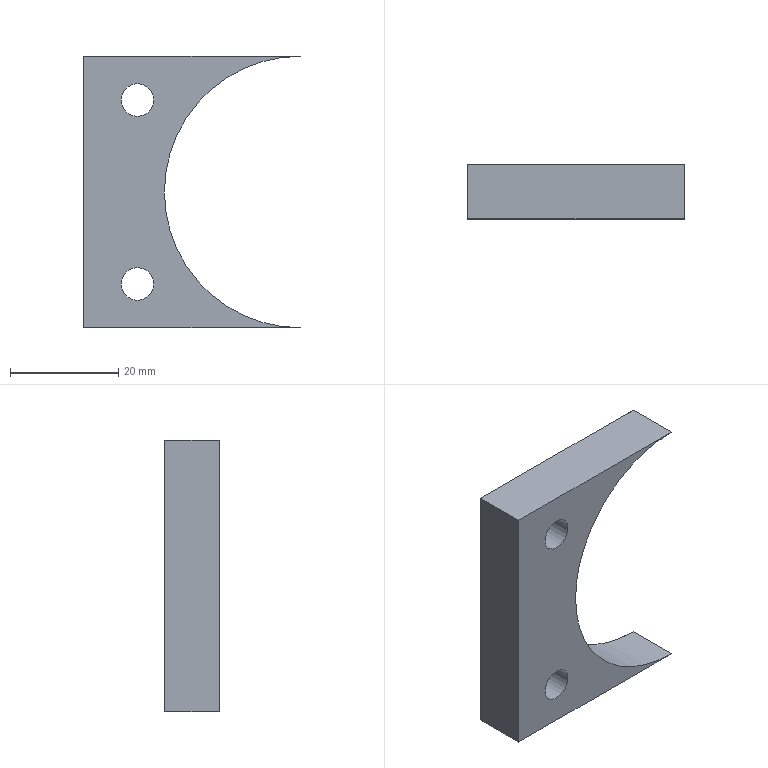Component | NX | GUIDEING_PLATE_2 | 1 solid | 10 faces | box 40 x 10 x 50.2 mm | volume 9461 mm3 | plane 5 | cylinder 3 | cone 2 | commonest cylinder face diameters 6 x2 50.2 x1
STEP:
#1=CARTESIAN_POINT('',(0.,0.,0.));
#2=DIRECTION('',(0.,0.,1.));
#3=DIRECTION('',(1.,0.,0.));
#4=AXIS2_PLACEMENT_3D('',#1,#2,#3);
#5=CARTESIAN_POINT('',(-114.9,110.,-25.1));
#6=VERTEX_POINT('',#5);
#7=CARTESIAN_POINT('',(-114.9,110.,25.1));
#8=VERTEX_POINT('',#7);
#9=CARTESIAN_POINT('',(-114.9,110.,-25.1));
#10=DIRECTION('',(0.,0.,1.));
#11=VECTOR('',#10,1.);
#12=LINE('',#9,#11);
#13=CARTESIAN_POINT('',(-114.9,120.,-25.1));
#14=DIRECTION('',(1.,0.,0.));
#15=DIRECTION('',(0.,-1.,0.));
#16=AXIS2_PLACEMENT_3D('',#13,#14,#15);
#17=PLANE('',#16);
#18=CARTESIAN_POINT('',(10.,0.));
#19=DIRECTION('',(0.,-1.));
#20=VECTOR('',#19,1.);
#21=LINE('',#18,#20);
#22=(GEOMETRIC_REPRESENTATION_CONTEXT(2)PARAMETRIC_REPRESENTATION_CONTEXT()REPRESENTATION_CONTEXT('',''));
#23=DEFINITIONAL_REPRESENTATION('',(#21),#22);
#24=PCURVE('',#17,#23);
#25=CARTESIAN_POINT('',(-74.9,110.,-0.));
#26=DIRECTION('',(0.,-1.,0.));
#27=DIRECTION('',(-1.,0.,0.));
#28=AXIS2_PLACEMENT_3D('',#25,#26,#27);
#29=PLANE('',#28);
#30=CARTESIAN_POINT('',(40.,25.1));
#31=DIRECTION('',(0.,-1.));
#32=VECTOR('',#31,1.);
#33=LINE('',#30,#32);
#34=(GEOMETRIC_REPRESENTATION_CONTEXT(2)PARAMETRIC_REPRESENTATION_CONTEXT()REPRESENTATION_CONTEXT('',''));
#35=DEFINITIONAL_REPRESENTATION('',(#33),#34);
#36=PCURVE('',#29,#35);
#37=SURFACE_CURVE('',#12,(#24,#36),.PCURVE_S1.);
#38=EDGE_CURVE('',#6,#8,#37,.T.);
#39=ORIENTED_EDGE('',*,*,#38,.T.);
#40=CARTESIAN_POINT('',(-114.9,120.,25.1));
#41=VERTEX_POINT('',#40);
#42=CARTESIAN_POINT('',(-114.9,120.,25.1));
#43=DIRECTION('',(0.,-1.,0.));
#44=VECTOR('',#43,1.);
#45=LINE('',#42,#44);
#46=CARTESIAN_POINT('',(0.,-50.2));
#47=DIRECTION('',(1.,0.));
#48=VECTOR('',#47,1.);
#49=LINE('',#46,#48);
#50=(GEOMETRIC_REPRESENTATION_CONTEXT(2)PARAMETRIC_REPRESENTATION_CONTEXT()REPRESENTATION_CONTEXT('',''));
#51=DEFINITIONAL_REPRESENTATION('',(#49),#50);
#52=PCURVE('',#17,#51);
#53=CARTESIAN_POINT('',(-114.9,120.,25.1));
#54=DIRECTION('',(0.,0.,-1.));
#55=DIRECTION('',(-1.,0.,-0.));
#56=AXIS2_PLACEMENT_3D('',#53,#54,#55);
#57=PLANE('',#56);
#58=CARTESIAN_POINT('',(0.,0.));
#59=DIRECTION('',(0.,-1.));
#60=VECTOR('',#59,1.);
#61=LINE('',#58,#60);
#62=(GEOMETRIC_REPRESENTATION_CONTEXT(2)PARAMETRIC_REPRESENTATION_CONTEXT()REPRESENTATION_CONTEXT('',''));
#63=DEFINITIONAL_REPRESENTATION('',(#61),#62);
#64=PCURVE('',#57,#63);
#65=SURFACE_CURVE('',#45,(#52,#64),.PCURVE_S1.);
#66=EDGE_CURVE('',#41,#8,#65,.T.);
#67=ORIENTED_EDGE('',*,*,#66,.F.);
#68=CARTESIAN_POINT('',(-114.9,120.,-25.1));
#69=VERTEX_POINT('',#68);
#70=CARTESIAN_POINT('',(-114.9,120.,-25.1));
#71=DIRECTION('',(0.,0.,1.));
#72=VECTOR('',#71,1.);
#73=LINE('',#70,#72);
#74=CARTESIAN_POINT('',(0.,0.));
#75=DIRECTION('',(0.,-1.));
#76=VECTOR('',#75,1.);
#77=LINE('',#74,#76);
#78=(GEOMETRIC_REPRESENTATION_CONTEXT(2)PARAMETRIC_REPRESENTATION_CONTEXT()REPRESENTATION_CONTEXT('',''));
#79=DEFINITIONAL_REPRESENTATION('',(#77),#78);
#80=PCURVE('',#17,#79);
#81=CARTESIAN_POINT('',(-74.9,120.,-0.));
#82=DIRECTION('',(0.,-1.,0.));
#83=DIRECTION('',(-1.,0.,0.));
#84=AXIS2_PLACEMENT_3D('',#81,#82,#83);
#85=PLANE('',#84);
#86=CARTESIAN_POINT('',(40.,25.1));
#87=DIRECTION('',(0.,-1.));
#88=VECTOR('',#87,1.);
#89=LINE('',#86,#88);
#90=(GEOMETRIC_REPRESENTATION_CONTEXT(2)PARAMETRIC_REPRESENTATION_CONTEXT()REPRESENTATION_CONTEXT('',''));
#91=DEFINITIONAL_REPRESENTATION('',(#89),#90);
#92=PCURVE('',#85,#91);
#93=SURFACE_CURVE('',#73,(#80,#92),.PCURVE_S1.);
#94=EDGE_CURVE('',#69,#41,#93,.T.);
#95=ORIENTED_EDGE('',*,*,#94,.F.);
#96=CARTESIAN_POINT('',(-114.9,120.,-25.1));
#97=DIRECTION('',(0.,-1.,0.));
#98=VECTOR('',#97,1.);
#99=LINE('',#96,#98);
#100=CARTESIAN_POINT('',(0.,0.));
#101=DIRECTION('',(1.,0.));
#102=VECTOR('',#101,1.);
#103=LINE('',#100,#102);
#104=(GEOMETRIC_REPRESENTATION_CONTEXT(2)PARAMETRIC_REPRESENTATION_CONTEXT()REPRESENTATION_CONTEXT('',''));
#105=DEFINITIONAL_REPRESENTATION('',(#103),#104);
#106=PCURVE('',#17,#105);
#107=CARTESIAN_POINT('',(-74.9,120.,-25.1));
#108=DIRECTION('',(0.,0.,1.));
#109=DIRECTION('',(1.,0.,-0.));
#110=AXIS2_PLACEMENT_3D('',#107,#108,#109);
#111=PLANE('',#110);
#112=CARTESIAN_POINT('',(-40.,0.));
#113=DIRECTION('',(0.,-1.));
#114=VECTOR('',#113,1.);
#115=LINE('',#112,#114);
#116=(GEOMETRIC_REPRESENTATION_CONTEXT(2)PARAMETRIC_REPRESENTATION_CONTEXT()REPRESENTATION_CONTEXT('',''));
#117=DEFINITIONAL_REPRESENTATION('',(#115),#116);
#118=PCURVE('',#111,#117);
#119=SURFACE_CURVE('',#99,(#106,#118),.PCURVE_S1.);
#120=EDGE_CURVE('',#69,#6,#119,.T.);
#121=ORIENTED_EDGE('',*,*,#120,.T.);
#122=EDGE_LOOP('',(#39,#67,#95,#121));
#123=FACE_BOUND('',#122,.T.);
#124=ADVANCED_FACE('',(#123),#17,.F.);
#125=CARTESIAN_POINT('',(-74.9,110.,25.1));
#126=VERTEX_POINT('',#125);
#127=CARTESIAN_POINT('',(-114.9,110.,25.1));
#128=DIRECTION('',(1.,0.,0.));
#129=VECTOR('',#128,1.);
#130=LINE('',#127,#129);
#131=CARTESIAN_POINT('',(0.,-10.));
#132=DIRECTION('',(-1.,0.));
#133=VECTOR('',#132,1.);
#134=LINE('',#131,#133);
#135=(GEOMETRIC_REPRESENTATION_CONTEXT(2)PARAMETRIC_REPRESENTATION_CONTEXT()REPRESENTATION_CONTEXT('',''));
#136=DEFINITIONAL_REPRESENTATION('',(#134),#135);
#137=PCURVE('',#57,#136);
#138=CARTESIAN_POINT('',(40.,-25.1));
#139=DIRECTION('',(-1.,-0.));
#140=VECTOR('',#139,1.);
#141=LINE('',#138,#140);
#142=(GEOMETRIC_REPRESENTATION_CONTEXT(2)PARAMETRIC_REPRESENTATION_CONTEXT()REPRESENTATION_CONTEXT('',''));
#143=DEFINITIONAL_REPRESENTATION('',(#141),#142);
#144=PCURVE('',#29,#143);
#145=SURFACE_CURVE('',#130,(#137,#144),.PCURVE_S1.);
#146=EDGE_CURVE('',#8,#126,#145,.T.);
#147=ORIENTED_EDGE('',*,*,#146,.T.);
#148=CARTESIAN_POINT('',(-74.9,120.,25.1));
#149=VERTEX_POINT('',#148);
#150=CARTESIAN_POINT('',(-74.9,120.,25.1));
#151=DIRECTION('',(0.,-1.,0.));
#152=VECTOR('',#151,1.);
#153=LINE('',#150,#152);
#154=CARTESIAN_POINT('',(-40.,0.));
#155=DIRECTION('',(0.,-1.));
#156=VECTOR('',#155,1.);
#157=LINE('',#154,#156);
#158=(GEOMETRIC_REPRESENTATION_CONTEXT(2)PARAMETRIC_REPRESENTATION_CONTEXT()REPRESENTATION_CONTEXT('',''));
#159=DEFINITIONAL_REPRESENTATION('',(#157),#158);
#160=PCURVE('',#57,#159);
#161=CARTESIAN_POINT('',(-74.9,120.,-0.));
#162=DIRECTION('',(0.,-1.,0.));
#163=DIRECTION('',(-1.,0.,0.));
#164=AXIS2_PLACEMENT_3D('',#161,#162,#163);
#165=CYLINDRICAL_SURFACE('',#164,25.1);
#166=CARTESIAN_POINT('',(4.712,0.));
#167=DIRECTION('',(0.,1.));
#168=VECTOR('',#167,1.);
#169=LINE('',#166,#168);
#170=(GEOMETRIC_REPRESENTATION_CONTEXT(2)PARAMETRIC_REPRESENTATION_CONTEXT()REPRESENTATION_CONTEXT('',''));
#171=DEFINITIONAL_REPRESENTATION('',(#169),#170);
#172=PCURVE('',#165,#171);
#173=SURFACE_CURVE('',#153,(#160,#172),.PCURVE_S1.);
#174=EDGE_CURVE('',#149,#126,#173,.T.);
#175=ORIENTED_EDGE('',*,*,#174,.F.);
#176=CARTESIAN_POINT('',(-114.9,120.,25.1));
#177=DIRECTION('',(1.,0.,0.));
#178=VECTOR('',#177,1.);
#179=LINE('',#176,#178);
#180=CARTESIAN_POINT('',(0.,0.));
#181=DIRECTION('',(-1.,0.));
#182=VECTOR('',#181,1.);
#183=LINE('',#180,#182);
#184=(GEOMETRIC_REPRESENTATION_CONTEXT(2)PARAMETRIC_REPRESENTATION_CONTEXT()REPRESENTATION_CONTEXT('',''));
#185=DEFINITIONAL_REPRESENTATION('',(#183),#184);
#186=PCURVE('',#57,#185);
#187=CARTESIAN_POINT('',(40.,-25.1));
#188=DIRECTION('',(-1.,-0.));
#189=VECTOR('',#188,1.);
#190=LINE('',#187,#189);
#191=(GEOMETRIC_REPRESENTATION_CONTEXT(2)PARAMETRIC_REPRESENTATION_CONTEXT()REPRESENTATION_CONTEXT('',''));
#192=DEFINITIONAL_REPRESENTATION('',(#190),#191);
#193=PCURVE('',#85,#192);
#194=SURFACE_CURVE('',#179,(#186,#193),.PCURVE_S1.);
#195=EDGE_CURVE('',#41,#149,#194,.T.);
#196=ORIENTED_EDGE('',*,*,#195,.F.);
#197=ORIENTED_EDGE('',*,*,#66,.T.);
#198=EDGE_LOOP('',(#147,#175,#196,#197));
#199=FACE_BOUND('',#198,.T.);
#200=ADVANCED_FACE('',(#199),#57,.F.);
#201=ORIENTED_EDGE('',*,*,#174,.F.);
#202=CARTESIAN_POINT('',(-74.9,120.,-25.1));
#203=VERTEX_POINT('',#202);
#204=CARTESIAN_POINT('',(-74.9,120.,-0.));
#205=DIRECTION('',(0.,-1.,0.));
#206=DIRECTION('',(1.,0.,-0.));
#207=AXIS2_PLACEMENT_3D('',#204,#205,#206);
#208=CIRCLE('',#207,25.1);
#209=CARTESIAN_POINT('',(3.142,0.));
#210=DIRECTION('',(1.,0.));
#211=VECTOR('',#210,1.);
#212=LINE('',#209,#211);
#213=(GEOMETRIC_REPRESENTATION_CONTEXT(2)PARAMETRIC_REPRESENTATION_CONTEXT()REPRESENTATION_CONTEXT('',''));
#214=DEFINITIONAL_REPRESENTATION('',(#212),#213);
#215=PCURVE('',#165,#214);
#216=CARTESIAN_POINT('',(0.,0.));
#217=DIRECTION('',(-1.,0.));
#218=AXIS2_PLACEMENT_2D('',#216,#217);
#219=CIRCLE('',#218,25.1);
#220=(GEOMETRIC_REPRESENTATION_CONTEXT(2)PARAMETRIC_REPRESENTATION_CONTEXT()REPRESENTATION_CONTEXT('',''));
#221=DEFINITIONAL_REPRESENTATION('',(#219),#220);
#222=PCURVE('',#85,#221);
#223=SURFACE_CURVE('',#208,(#215,#222),.PCURVE_S1.);
#224=EDGE_CURVE('',#149,#203,#223,.T.);
#225=ORIENTED_EDGE('',*,*,#224,.T.);
#226=CARTESIAN_POINT('',(-74.9,110.,-25.1));
#227=VERTEX_POINT('',#226);
#228=CARTESIAN_POINT('',(-74.9,120.,-25.1));
#229=DIRECTION('',(0.,-1.,0.));
#230=VECTOR('',#229,1.);
#231=LINE('',#228,#230);
#232=CARTESIAN_POINT('',(7.854,0.));
#233=DIRECTION('',(0.,1.));
#234=VECTOR('',#233,1.);
#235=LINE('',#232,#234);
#236=(GEOMETRIC_REPRESENTATION_CONTEXT(2)PARAMETRIC_REPRESENTATION_CONTEXT()REPRESENTATION_CONTEXT('',''));
#237=DEFINITIONAL_REPRESENTATION('',(#235),#236);
#238=PCURVE('',#165,#237);
#239=CARTESIAN_POINT('',(0.,0.));
#240=DIRECTION('',(0.,-1.));
#241=VECTOR('',#240,1.);
#242=LINE('',#239,#241);
#243=(GEOMETRIC_REPRESENTATION_CONTEXT(2)PARAMETRIC_REPRESENTATION_CONTEXT()REPRESENTATION_CONTEXT('',''));
#244=DEFINITIONAL_REPRESENTATION('',(#242),#243);
#245=PCURVE('',#111,#244);
#246=SURFACE_CURVE('',#231,(#238,#245),.PCURVE_S1.);
#247=EDGE_CURVE('',#203,#227,#246,.T.);
#248=ORIENTED_EDGE('',*,*,#247,.T.);
#249=CARTESIAN_POINT('',(-74.9,110.,-0.));
#250=DIRECTION('',(0.,-1.,0.));
#251=DIRECTION('',(1.,0.,-0.));
#252=AXIS2_PLACEMENT_3D('',#249,#250,#251);
#253=CIRCLE('',#252,25.1);
#254=CARTESIAN_POINT('',(3.142,10.));
#255=DIRECTION('',(1.,0.));
#256=VECTOR('',#255,1.);
#257=LINE('',#254,#256);
#258=(GEOMETRIC_REPRESENTATION_CONTEXT(2)PARAMETRIC_REPRESENTATION_CONTEXT()REPRESENTATION_CONTEXT('',''));
#259=DEFINITIONAL_REPRESENTATION('',(#257),#258);
#260=PCURVE('',#165,#259);
#261=CARTESIAN_POINT('',(0.,0.));
#262=DIRECTION('',(-1.,0.));
#263=AXIS2_PLACEMENT_2D('',#261,#262);
#264=CIRCLE('',#263,25.1);
#265=(GEOMETRIC_REPRESENTATION_CONTEXT(2)PARAMETRIC_REPRESENTATION_CONTEXT()REPRESENTATION_CONTEXT('',''));
#266=DEFINITIONAL_REPRESENTATION('',(#264),#265);
#267=PCURVE('',#29,#266);
#268=SURFACE_CURVE('',#253,(#260,#267),.PCURVE_S1.);
#269=EDGE_CURVE('',#126,#227,#268,.T.);
#270=ORIENTED_EDGE('',*,*,#269,.F.);
#271=EDGE_LOOP('',(#201,#225,#248,#270));
#272=FACE_BOUND('',#271,.F.);
#273=ADVANCED_FACE('',(#272),#165,.F.);
#274=CARTESIAN_POINT('',(-74.9,110.,-25.1));
#275=DIRECTION('',(-1.,0.,0.));
#276=VECTOR('',#275,1.);
#277=LINE('',#274,#276);
#278=CARTESIAN_POINT('',(0.,-10.));
#279=DIRECTION('',(-1.,0.));
#280=VECTOR('',#279,1.);
#281=LINE('',#278,#280);
#282=(GEOMETRIC_REPRESENTATION_CONTEXT(2)PARAMETRIC_REPRESENTATION_CONTEXT()REPRESENTATION_CONTEXT('',''));
#283=DEFINITIONAL_REPRESENTATION('',(#281),#282);
#284=PCURVE('',#111,#283);
#285=CARTESIAN_POINT('',(0.,25.1));
#286=DIRECTION('',(1.,-0.));
#287=VECTOR('',#286,1.);
#288=LINE('',#285,#287);
#289=(GEOMETRIC_REPRESENTATION_CONTEXT(2)PARAMETRIC_REPRESENTATION_CONTEXT()REPRESENTATION_CONTEXT('',''));
#290=DEFINITIONAL_REPRESENTATION('',(#288),#289);
#291=PCURVE('',#29,#290);
#292=SURFACE_CURVE('',#277,(#284,#291),.PCURVE_S1.);
#293=EDGE_CURVE('',#227,#6,#292,.T.);
#294=ORIENTED_EDGE('',*,*,#293,.T.);
#295=ORIENTED_EDGE('',*,*,#120,.F.);
#296=CARTESIAN_POINT('',(-74.9,120.,-25.1));
#297=DIRECTION('',(-1.,0.,0.));
#298=VECTOR('',#297,1.);
#299=LINE('',#296,#298);
#300=CARTESIAN_POINT('',(0.,0.));
#301=DIRECTION('',(-1.,0.));
#302=VECTOR('',#301,1.);
#303=LINE('',#300,#302);
#304=(GEOMETRIC_REPRESENTATION_CONTEXT(2)PARAMETRIC_REPRESENTATION_CONTEXT()REPRESENTATION_CONTEXT('',''));
#305=DEFINITIONAL_REPRESENTATION('',(#303),#304);
#306=PCURVE('',#111,#305);
#307=CARTESIAN_POINT('',(0.,25.1));
#308=DIRECTION('',(1.,-0.));
#309=VECTOR('',#308,1.);
#310=LINE('',#307,#309);
#311=(GEOMETRIC_REPRESENTATION_CONTEXT(2)PARAMETRIC_REPRESENTATION_CONTEXT()REPRESENTATION_CONTEXT('',''));
#312=DEFINITIONAL_REPRESENTATION('',(#310),#311);
#313=PCURVE('',#85,#312);
#314=SURFACE_CURVE('',#299,(#306,#313),.PCURVE_S1.);
#315=EDGE_CURVE('',#203,#69,#314,.T.);
#316=ORIENTED_EDGE('',*,*,#315,.F.);
#317=ORIENTED_EDGE('',*,*,#247,.T.);
#318=EDGE_LOOP('',(#294,#295,#316,#317));
#319=FACE_BOUND('',#318,.T.);
#320=ADVANCED_FACE('',(#319),#111,.F.);
#321=CARTESIAN_POINT('',(-110.55,120.,17.));
#322=VERTEX_POINT('',#321);
#323=CARTESIAN_POINT('',(-105.,120.,17.));
#324=DIRECTION('',(0.,-1.,0.));
#325=DIRECTION('',(-1.,0.,0.));
#326=AXIS2_PLACEMENT_3D('',#323,#324,#325);
#327=CIRCLE('',#326,5.55);
#328=CARTESIAN_POINT('',(30.1,-17.));
#329=DIRECTION('',(1.,0.));
#330=AXIS2_PLACEMENT_2D('',#328,#329);
#331=CIRCLE('',#330,5.55);
#332=(GEOMETRIC_REPRESENTATION_CONTEXT(2)PARAMETRIC_REPRESENTATION_CONTEXT()REPRESENTATION_CONTEXT('',''));
#333=DEFINITIONAL_REPRESENTATION('',(#331),#332);
#334=PCURVE('',#85,#333);
#335=CARTESIAN_POINT('',(-105.,120.,17.));
#336=DIRECTION('',(0.,1.,0.));
#337=DIRECTION('',(1.,0.,0.));
#338=AXIS2_PLACEMENT_3D('',#335,#336,#337);
#339=CONICAL_SURFACE('',#338,5.55,0.7854);
#340=CARTESIAN_POINT('',(9.425,-0.));
#341=DIRECTION('',(-1.,0.));
#342=VECTOR('',#341,1.);
#343=LINE('',#340,#342);
#344=(GEOMETRIC_REPRESENTATION_CONTEXT(2)PARAMETRIC_REPRESENTATION_CONTEXT()REPRESENTATION_CONTEXT('',''));
#345=DEFINITIONAL_REPRESENTATION('',(#343),#344);
#346=PCURVE('',#339,#345);
#347=SURFACE_CURVE('',#327,(#334,#346),.PCURVE_S1.);
#348=EDGE_CURVE('',#322,#322,#347,.T.);
#349=ORIENTED_EDGE('',*,*,#348,.T.);
#350=EDGE_LOOP('',(#349));
#351=FACE_BOUND('',#350,.T.);
#352=CARTESIAN_POINT('',(-110.55,120.,-17.));
#353=VERTEX_POINT('',#352);
#354=CARTESIAN_POINT('',(-105.,120.,-17.));
#355=DIRECTION('',(0.,-1.,0.));
#356=DIRECTION('',(-1.,0.,0.));
#357=AXIS2_PLACEMENT_3D('',#354,#355,#356);
#358=CIRCLE('',#357,5.55);
#359=CARTESIAN_POINT('',(30.1,17.));
#360=DIRECTION('',(1.,0.));
#361=AXIS2_PLACEMENT_2D('',#359,#360);
#362=CIRCLE('',#361,5.55);
#363=(GEOMETRIC_REPRESENTATION_CONTEXT(2)PARAMETRIC_REPRESENTATION_CONTEXT()REPRESENTATION_CONTEXT('',''));
#364=DEFINITIONAL_REPRESENTATION('',(#362),#363);
#365=PCURVE('',#85,#364);
#366=CARTESIAN_POINT('',(-105.,120.,-17.));
#367=DIRECTION('',(0.,1.,0.));
#368=DIRECTION('',(1.,0.,0.));
#369=AXIS2_PLACEMENT_3D('',#366,#367,#368);
#370=CONICAL_SURFACE('',#369,5.55,0.7854);
#371=CARTESIAN_POINT('',(9.425,-0.));
#372=DIRECTION('',(-1.,0.));
#373=VECTOR('',#372,1.);
#374=LINE('',#371,#373);
#375=(GEOMETRIC_REPRESENTATION_CONTEXT(2)PARAMETRIC_REPRESENTATION_CONTEXT()REPRESENTATION_CONTEXT('',''));
#376=DEFINITIONAL_REPRESENTATION('',(#374),#375);
#377=PCURVE('',#370,#376);
#378=SURFACE_CURVE('',#358,(#365,#377),.PCURVE_S1.);
#379=EDGE_CURVE('',#353,#353,#378,.T.);
#380=ORIENTED_EDGE('',*,*,#379,.T.);
#381=EDGE_LOOP('',(#380));
#382=FACE_BOUND('',#381,.T.);
#383=ORIENTED_EDGE('',*,*,#94,.T.);
#384=ORIENTED_EDGE('',*,*,#195,.T.);
#385=ORIENTED_EDGE('',*,*,#224,.T.);
#386=ORIENTED_EDGE('',*,*,#315,.T.);
#387=EDGE_LOOP('',(#383,#384,#385,#386));
#388=FACE_BOUND('',#387,.T.);
#389=ADVANCED_FACE('',(#351,#382,#388),#85,.F.);
#390=CARTESIAN_POINT('',(-108.,110.,17.));
#391=VERTEX_POINT('',#390);
#392=CARTESIAN_POINT('',(-105.,110.,17.));
#393=DIRECTION('',(0.,-1.,0.));
#394=DIRECTION('',(-1.,0.,0.));
#395=AXIS2_PLACEMENT_3D('',#392,#393,#394);
#396=CIRCLE('',#395,3.);
#397=CARTESIAN_POINT('',(30.1,-17.));
#398=DIRECTION('',(1.,0.));
#399=AXIS2_PLACEMENT_2D('',#397,#398);
#400=CIRCLE('',#399,3.);
#401=(GEOMETRIC_REPRESENTATION_CONTEXT(2)PARAMETRIC_REPRESENTATION_CONTEXT()REPRESENTATION_CONTEXT('',''));
#402=DEFINITIONAL_REPRESENTATION('',(#400),#401);
#403=PCURVE('',#29,#402);
#404=CARTESIAN_POINT('',(-105.,-494884.989,17.));
#405=DIRECTION('',(0.,-1.,0.));
#406=DIRECTION('',(-1.,0.,0.));
#407=AXIS2_PLACEMENT_3D('',#404,#405,#406);
#408=CYLINDRICAL_SURFACE('',#407,3.);
#409=CARTESIAN_POINT('',(0.,-494994.989));
#410=DIRECTION('',(1.,0.));
#411=VECTOR('',#410,1.);
#412=LINE('',#409,#411);
#413=(GEOMETRIC_REPRESENTATION_CONTEXT(2)PARAMETRIC_REPRESENTATION_CONTEXT()REPRESENTATION_CONTEXT('',''));
#414=DEFINITIONAL_REPRESENTATION('',(#412),#413);
#415=PCURVE('',#408,#414);
#416=SURFACE_CURVE('',#396,(#403,#415),.PCURVE_S1.);
#417=EDGE_CURVE('',#391,#391,#416,.T.);
#418=ORIENTED_EDGE('',*,*,#417,.F.);
#419=EDGE_LOOP('',(#418));
#420=FACE_BOUND('',#419,.T.);
#421=CARTESIAN_POINT('',(-108.,110.,-17.));
#422=VERTEX_POINT('',#421);
#423=CARTESIAN_POINT('',(-105.,110.,-17.));
#424=DIRECTION('',(0.,-1.,0.));
#425=DIRECTION('',(-1.,0.,0.));
#426=AXIS2_PLACEMENT_3D('',#423,#424,#425);
#427=CIRCLE('',#426,3.);
#428=CARTESIAN_POINT('',(30.1,17.));
#429=DIRECTION('',(1.,0.));
#430=AXIS2_PLACEMENT_2D('',#428,#429);
#431=CIRCLE('',#430,3.);
#432=(GEOMETRIC_REPRESENTATION_CONTEXT(2)PARAMETRIC_REPRESENTATION_CONTEXT()REPRESENTATION_CONTEXT('',''));
#433=DEFINITIONAL_REPRESENTATION('',(#431),#432);
#434=PCURVE('',#29,#433);
#435=CARTESIAN_POINT('',(-105.,-494884.989,-17.));
#436=DIRECTION('',(0.,-1.,0.));
#437=DIRECTION('',(-1.,0.,0.));
#438=AXIS2_PLACEMENT_3D('',#435,#436,#437);
#439=CYLINDRICAL_SURFACE('',#438,3.);
#440=CARTESIAN_POINT('',(0.,-494994.989));
#441=DIRECTION('',(1.,0.));
#442=VECTOR('',#441,1.);
#443=LINE('',#440,#442);
#444=(GEOMETRIC_REPRESENTATION_CONTEXT(2)PARAMETRIC_REPRESENTATION_CONTEXT()REPRESENTATION_CONTEXT('',''));
#445=DEFINITIONAL_REPRESENTATION('',(#443),#444);
#446=PCURVE('',#439,#445);
#447=SURFACE_CURVE('',#427,(#434,#446),.PCURVE_S1.);
#448=EDGE_CURVE('',#422,#422,#447,.T.);
#449=ORIENTED_EDGE('',*,*,#448,.F.);
#450=EDGE_LOOP('',(#449));
#451=FACE_BOUND('',#450,.T.);
#452=ORIENTED_EDGE('',*,*,#38,.F.);
#453=ORIENTED_EDGE('',*,*,#293,.F.);
#454=ORIENTED_EDGE('',*,*,#269,.F.);
#455=ORIENTED_EDGE('',*,*,#146,.F.);
#456=EDGE_LOOP('',(#452,#453,#454,#455));
#457=FACE_BOUND('',#456,.T.);
#458=ADVANCED_FACE('',(#420,#451,#457),#29,.T.);
#459=ORIENTED_EDGE('',*,*,#448,.F.);
#460=CARTESIAN_POINT('',(-108.,117.45,-17.));
#461=VERTEX_POINT('',#460);
#462=CARTESIAN_POINT('',(-108.,117.45,-17.));
#463=CARTESIAN_POINT('',(-108.,110.,-17.));
#464=B_SPLINE_CURVE_WITH_KNOTS('',1,(#462,#463),.UNSPECIFIED.,.F.,.F.,(2,2),(-495002.439,-494994.989),.PIECEWISE_BEZIER_KNOTS.);
#465=CARTESIAN_POINT('',(0.,0.));
#466=DIRECTION('',(0.,1.));
#467=VECTOR('',#466,1.);
#468=LINE('',#465,#467);
#469=(GEOMETRIC_REPRESENTATION_CONTEXT(2)PARAMETRIC_REPRESENTATION_CONTEXT()REPRESENTATION_CONTEXT('',''));
#470=DEFINITIONAL_REPRESENTATION('',(#468),#469);
#471=PCURVE('',#439,#470);
#472=CARTESIAN_POINT('',(6.283,0.));
#473=DIRECTION('',(0.,1.));
#474=VECTOR('',#473,1.);
#475=LINE('',#472,#474);
#476=(GEOMETRIC_REPRESENTATION_CONTEXT(2)PARAMETRIC_REPRESENTATION_CONTEXT()REPRESENTATION_CONTEXT('',''));
#477=DEFINITIONAL_REPRESENTATION('',(#475),#476);
#478=PCURVE('',#439,#477);
#479=SEAM_CURVE('',#464,(#471,#478),.PCURVE_S1.);
#480=EDGE_CURVE('',#461,#422,#479,.T.);
#481=ORIENTED_EDGE('',*,*,#480,.F.);
#482=CARTESIAN_POINT('',(-105.,117.45,-17.));
#483=DIRECTION('',(0.,1.,0.));
#484=DIRECTION('',(-1.,0.,0.));
#485=AXIS2_PLACEMENT_3D('',#482,#483,#484);
#486=CIRCLE('',#485,3.);
#487=CARTESIAN_POINT('',(6.283,-495002.439));
#488=DIRECTION('',(-1.,0.));
#489=VECTOR('',#488,1.);
#490=LINE('',#487,#489);
#491=(GEOMETRIC_REPRESENTATION_CONTEXT(2)PARAMETRIC_REPRESENTATION_CONTEXT()REPRESENTATION_CONTEXT('',''));
#492=DEFINITIONAL_REPRESENTATION('',(#490),#491);
#493=PCURVE('',#439,#492);
#494=CARTESIAN_POINT('',(3.142,-2.55));
#495=DIRECTION('',(1.,0.));
#496=VECTOR('',#495,1.);
#497=LINE('',#494,#496);
#498=(GEOMETRIC_REPRESENTATION_CONTEXT(2)PARAMETRIC_REPRESENTATION_CONTEXT()REPRESENTATION_CONTEXT('',''));
#499=DEFINITIONAL_REPRESENTATION('',(#497),#498);
#500=PCURVE('',#370,#499);
#501=SURFACE_CURVE('',#486,(#493,#500),.PCURVE_S1.);
#502=EDGE_CURVE('',#461,#461,#501,.T.);
#503=ORIENTED_EDGE('',*,*,#502,.F.);
#504=ORIENTED_EDGE('',*,*,#480,.T.);
#505=EDGE_LOOP('',(#459,#481,#503,#504));
#506=FACE_BOUND('',#505,.F.);
#507=ADVANCED_FACE('',(#506),#439,.F.);
#508=ORIENTED_EDGE('',*,*,#502,.T.);
#509=CARTESIAN_POINT('',(-108.,117.45,-17.));
#510=CARTESIAN_POINT('',(-110.55,120.,-17.));
#511=B_SPLINE_CURVE_WITH_KNOTS('',1,(#509,#510),.UNSPECIFIED.,.F.,.F.,(2,2),(-3.606,-0.),.PIECEWISE_BEZIER_KNOTS.);
#512=CARTESIAN_POINT('',(9.425,0.));
#513=DIRECTION('',(0.,1.));
#514=VECTOR('',#513,1.);
#515=LINE('',#512,#514);
#516=(GEOMETRIC_REPRESENTATION_CONTEXT(2)PARAMETRIC_REPRESENTATION_CONTEXT()REPRESENTATION_CONTEXT('',''));
#517=DEFINITIONAL_REPRESENTATION('',(#515),#516);
#518=PCURVE('',#370,#517);
#519=CARTESIAN_POINT('',(3.142,0.));
#520=DIRECTION('',(0.,1.));
#521=VECTOR('',#520,1.);
#522=LINE('',#519,#521);
#523=(GEOMETRIC_REPRESENTATION_CONTEXT(2)PARAMETRIC_REPRESENTATION_CONTEXT()REPRESENTATION_CONTEXT('',''));
#524=DEFINITIONAL_REPRESENTATION('',(#522),#523);
#525=PCURVE('',#370,#524);
#526=SEAM_CURVE('',#511,(#518,#525),.PCURVE_S1.);
#527=EDGE_CURVE('',#461,#353,#526,.T.);
#528=ORIENTED_EDGE('',*,*,#527,.T.);
#529=ORIENTED_EDGE('',*,*,#379,.T.);
#530=ORIENTED_EDGE('',*,*,#527,.F.);
#531=EDGE_LOOP('',(#508,#528,#529,#530));
#532=FACE_BOUND('',#531,.F.);
#533=ADVANCED_FACE('',(#532),#370,.F.);
#534=ORIENTED_EDGE('',*,*,#417,.F.);
#535=CARTESIAN_POINT('',(-108.,117.45,17.));
#536=VERTEX_POINT('',#535);
#537=CARTESIAN_POINT('',(-108.,117.45,17.));
#538=CARTESIAN_POINT('',(-108.,110.,17.));
#539=B_SPLINE_CURVE_WITH_KNOTS('',1,(#537,#538),.UNSPECIFIED.,.F.,.F.,(2,2),(-495002.439,-494994.989),.PIECEWISE_BEZIER_KNOTS.);
#540=CARTESIAN_POINT('',(0.,0.));
#541=DIRECTION('',(0.,1.));
#542=VECTOR('',#541,1.);
#543=LINE('',#540,#542);
#544=(GEOMETRIC_REPRESENTATION_CONTEXT(2)PARAMETRIC_REPRESENTATION_CONTEXT()REPRESENTATION_CONTEXT('',''));
#545=DEFINITIONAL_REPRESENTATION('',(#543),#544);
#546=PCURVE('',#408,#545);
#547=CARTESIAN_POINT('',(6.283,0.));
#548=DIRECTION('',(0.,1.));
#549=VECTOR('',#548,1.);
#550=LINE('',#547,#549);
#551=(GEOMETRIC_REPRESENTATION_CONTEXT(2)PARAMETRIC_REPRESENTATION_CONTEXT()REPRESENTATION_CONTEXT('',''));
#552=DEFINITIONAL_REPRESENTATION('',(#550),#551);
#553=PCURVE('',#408,#552);
#554=SEAM_CURVE('',#539,(#546,#553),.PCURVE_S1.);
#555=EDGE_CURVE('',#536,#391,#554,.T.);
#556=ORIENTED_EDGE('',*,*,#555,.F.);
#557=CARTESIAN_POINT('',(-105.,117.45,17.));
#558=DIRECTION('',(0.,1.,0.));
#559=DIRECTION('',(-1.,0.,0.));
#560=AXIS2_PLACEMENT_3D('',#557,#558,#559);
#561=CIRCLE('',#560,3.);
#562=CARTESIAN_POINT('',(6.283,-495002.439));
#563=DIRECTION('',(-1.,0.));
#564=VECTOR('',#563,1.);
#565=LINE('',#562,#564);
#566=(GEOMETRIC_REPRESENTATION_CONTEXT(2)PARAMETRIC_REPRESENTATION_CONTEXT()REPRESENTATION_CONTEXT('',''));
#567=DEFINITIONAL_REPRESENTATION('',(#565),#566);
#568=PCURVE('',#408,#567);
#569=CARTESIAN_POINT('',(3.142,-2.55));
#570=DIRECTION('',(1.,0.));
#571=VECTOR('',#570,1.);
#572=LINE('',#569,#571);
#573=(GEOMETRIC_REPRESENTATION_CONTEXT(2)PARAMETRIC_REPRESENTATION_CONTEXT()REPRESENTATION_CONTEXT('',''));
#574=DEFINITIONAL_REPRESENTATION('',(#572),#573);
#575=PCURVE('',#339,#574);
#576=SURFACE_CURVE('',#561,(#568,#575),.PCURVE_S1.);
#577=EDGE_CURVE('',#536,#536,#576,.T.);
#578=ORIENTED_EDGE('',*,*,#577,.F.);
#579=ORIENTED_EDGE('',*,*,#555,.T.);
#580=EDGE_LOOP('',(#534,#556,#578,#579));
#581=FACE_BOUND('',#580,.F.);
#582=ADVANCED_FACE('',(#581),#408,.F.);
#583=ORIENTED_EDGE('',*,*,#577,.T.);
#584=CARTESIAN_POINT('',(-108.,117.45,17.));
#585=CARTESIAN_POINT('',(-110.55,120.,17.));
#586=B_SPLINE_CURVE_WITH_KNOTS('',1,(#584,#585),.UNSPECIFIED.,.F.,.F.,(2,2),(-3.606,-0.),.PIECEWISE_BEZIER_KNOTS.);
#587=CARTESIAN_POINT('',(9.425,0.));
#588=DIRECTION('',(0.,1.));
#589=VECTOR('',#588,1.);
#590=LINE('',#587,#589);
#591=(GEOMETRIC_REPRESENTATION_CONTEXT(2)PARAMETRIC_REPRESENTATION_CONTEXT()REPRESENTATION_CONTEXT('',''));
#592=DEFINITIONAL_REPRESENTATION('',(#590),#591);
#593=PCURVE('',#339,#592);
#594=CARTESIAN_POINT('',(3.142,0.));
#595=DIRECTION('',(0.,1.));
#596=VECTOR('',#595,1.);
#597=LINE('',#594,#596);
#598=(GEOMETRIC_REPRESENTATION_CONTEXT(2)PARAMETRIC_REPRESENTATION_CONTEXT()REPRESENTATION_CONTEXT('',''));
#599=DEFINITIONAL_REPRESENTATION('',(#597),#598);
#600=PCURVE('',#339,#599);
#601=SEAM_CURVE('',#586,(#593,#600),.PCURVE_S1.);
#602=EDGE_CURVE('',#536,#322,#601,.T.);
#603=ORIENTED_EDGE('',*,*,#602,.T.);
#604=ORIENTED_EDGE('',*,*,#348,.T.);
#605=ORIENTED_EDGE('',*,*,#602,.F.);
#606=EDGE_LOOP('',(#583,#603,#604,#605));
#607=FACE_BOUND('',#606,.F.);
#608=ADVANCED_FACE('',(#607),#339,.F.);
#609=CLOSED_SHELL('',(#124,#200,#273,#320,#389,#458,#507,#533,#582,#608));
#610=MANIFOLD_SOLID_BREP('',#609);
#611=(LENGTH_UNIT()NAMED_UNIT(*)SI_UNIT(.MILLI.,.METRE.));
#612=UNCERTAINTY_MEASURE_WITH_UNIT(LENGTH_MEASURE(0.000005),#611,'','');
#613=(NAMED_UNIT(*)PLANE_ANGLE_UNIT()SI_UNIT($,.RADIAN.));
#614=(NAMED_UNIT(*)SI_UNIT($,.STERADIAN.)SOLID_ANGLE_UNIT());
#615=(GEOMETRIC_REPRESENTATION_CONTEXT(3)GLOBAL_UNCERTAINTY_ASSIGNED_CONTEXT((#612))GLOBAL_UNIT_ASSIGNED_CONTEXT((#611,#613,#614))REPRESENTATION_CONTEXT('',''));
#616=ADVANCED_BREP_SHAPE_REPRESENTATION('',(#4,#610),#615);